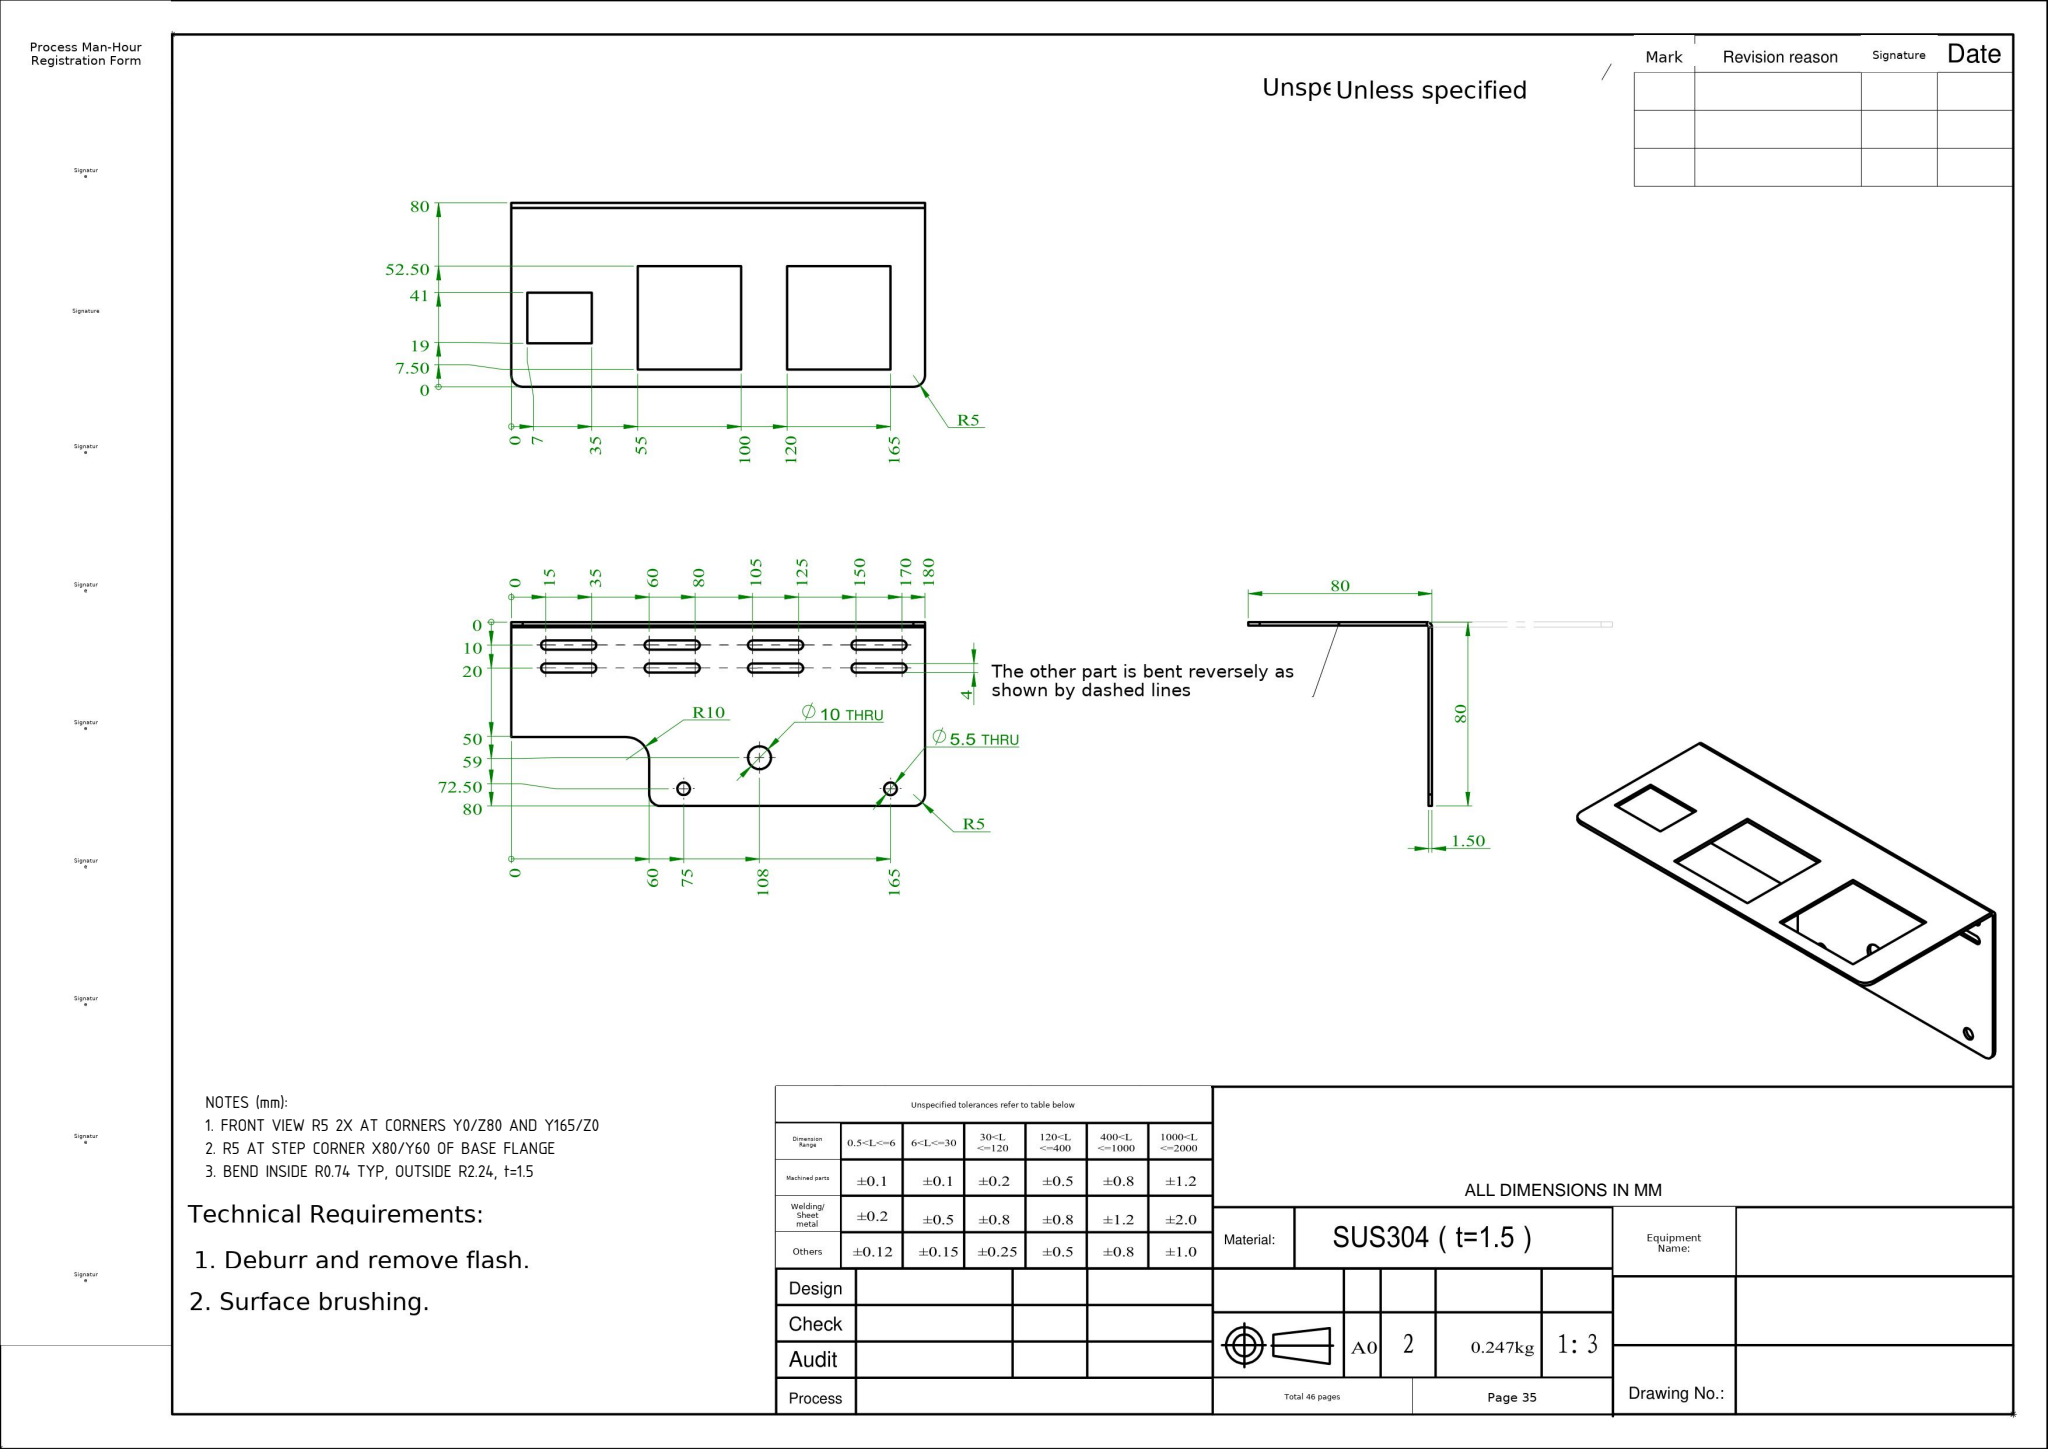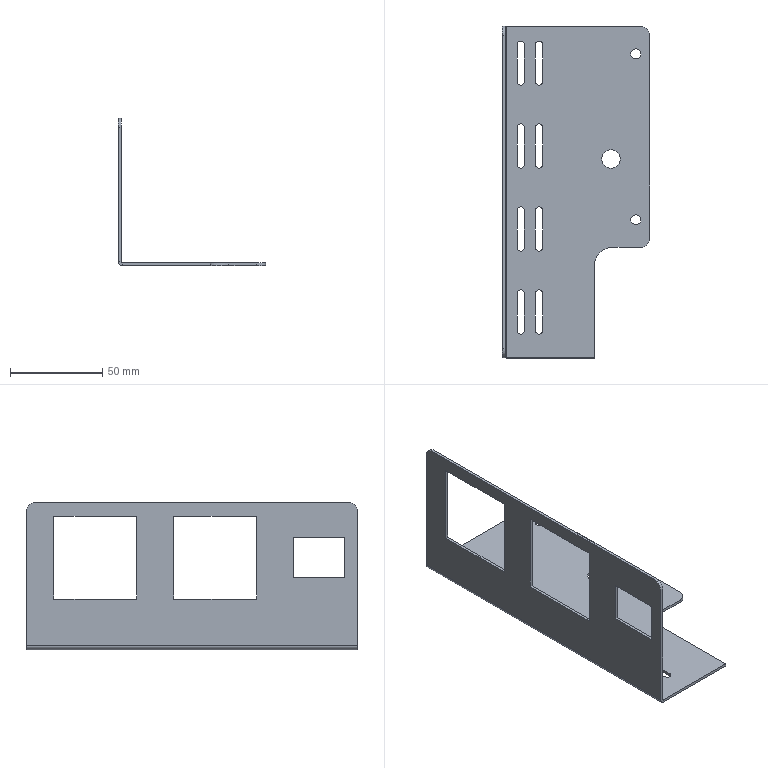Part | SolidWorks | mm | 1 solid | 71 faces | box 80 x 180 x 80 mm | volume 31624 mm3 | plane 42 | cylinder 29 | commonest cylinder face diameters 4 x16 10 x6 5.5 x4 4.473 x1 1.473 x1 20 x1
Drawing notes:
FRONT VIEW R5 2X AT CORNERS Y0/Z80 AND Y165/Z0 | from the solid: Vert face (x=0..1.5) 180x80 outline shows 5mm corner breaks at Y0/Z80 and Y165/Z0
R5 AT STEP CORNER X80/Y60 OF BASE FLANGE | from the solid: cyl dia 10.0 axis z at (x=75, y=65), len 1.5 -> R5 convex corner at x=80, y=60
BEND INSIDE R0.74 TYP, OUTSIDE R2.24, t=1.5 | from the solid: cyl dia 1.473 axis y at (2.24,2.24) L180 = inner R0.74; dia 4.473 same axis = outer R2.24